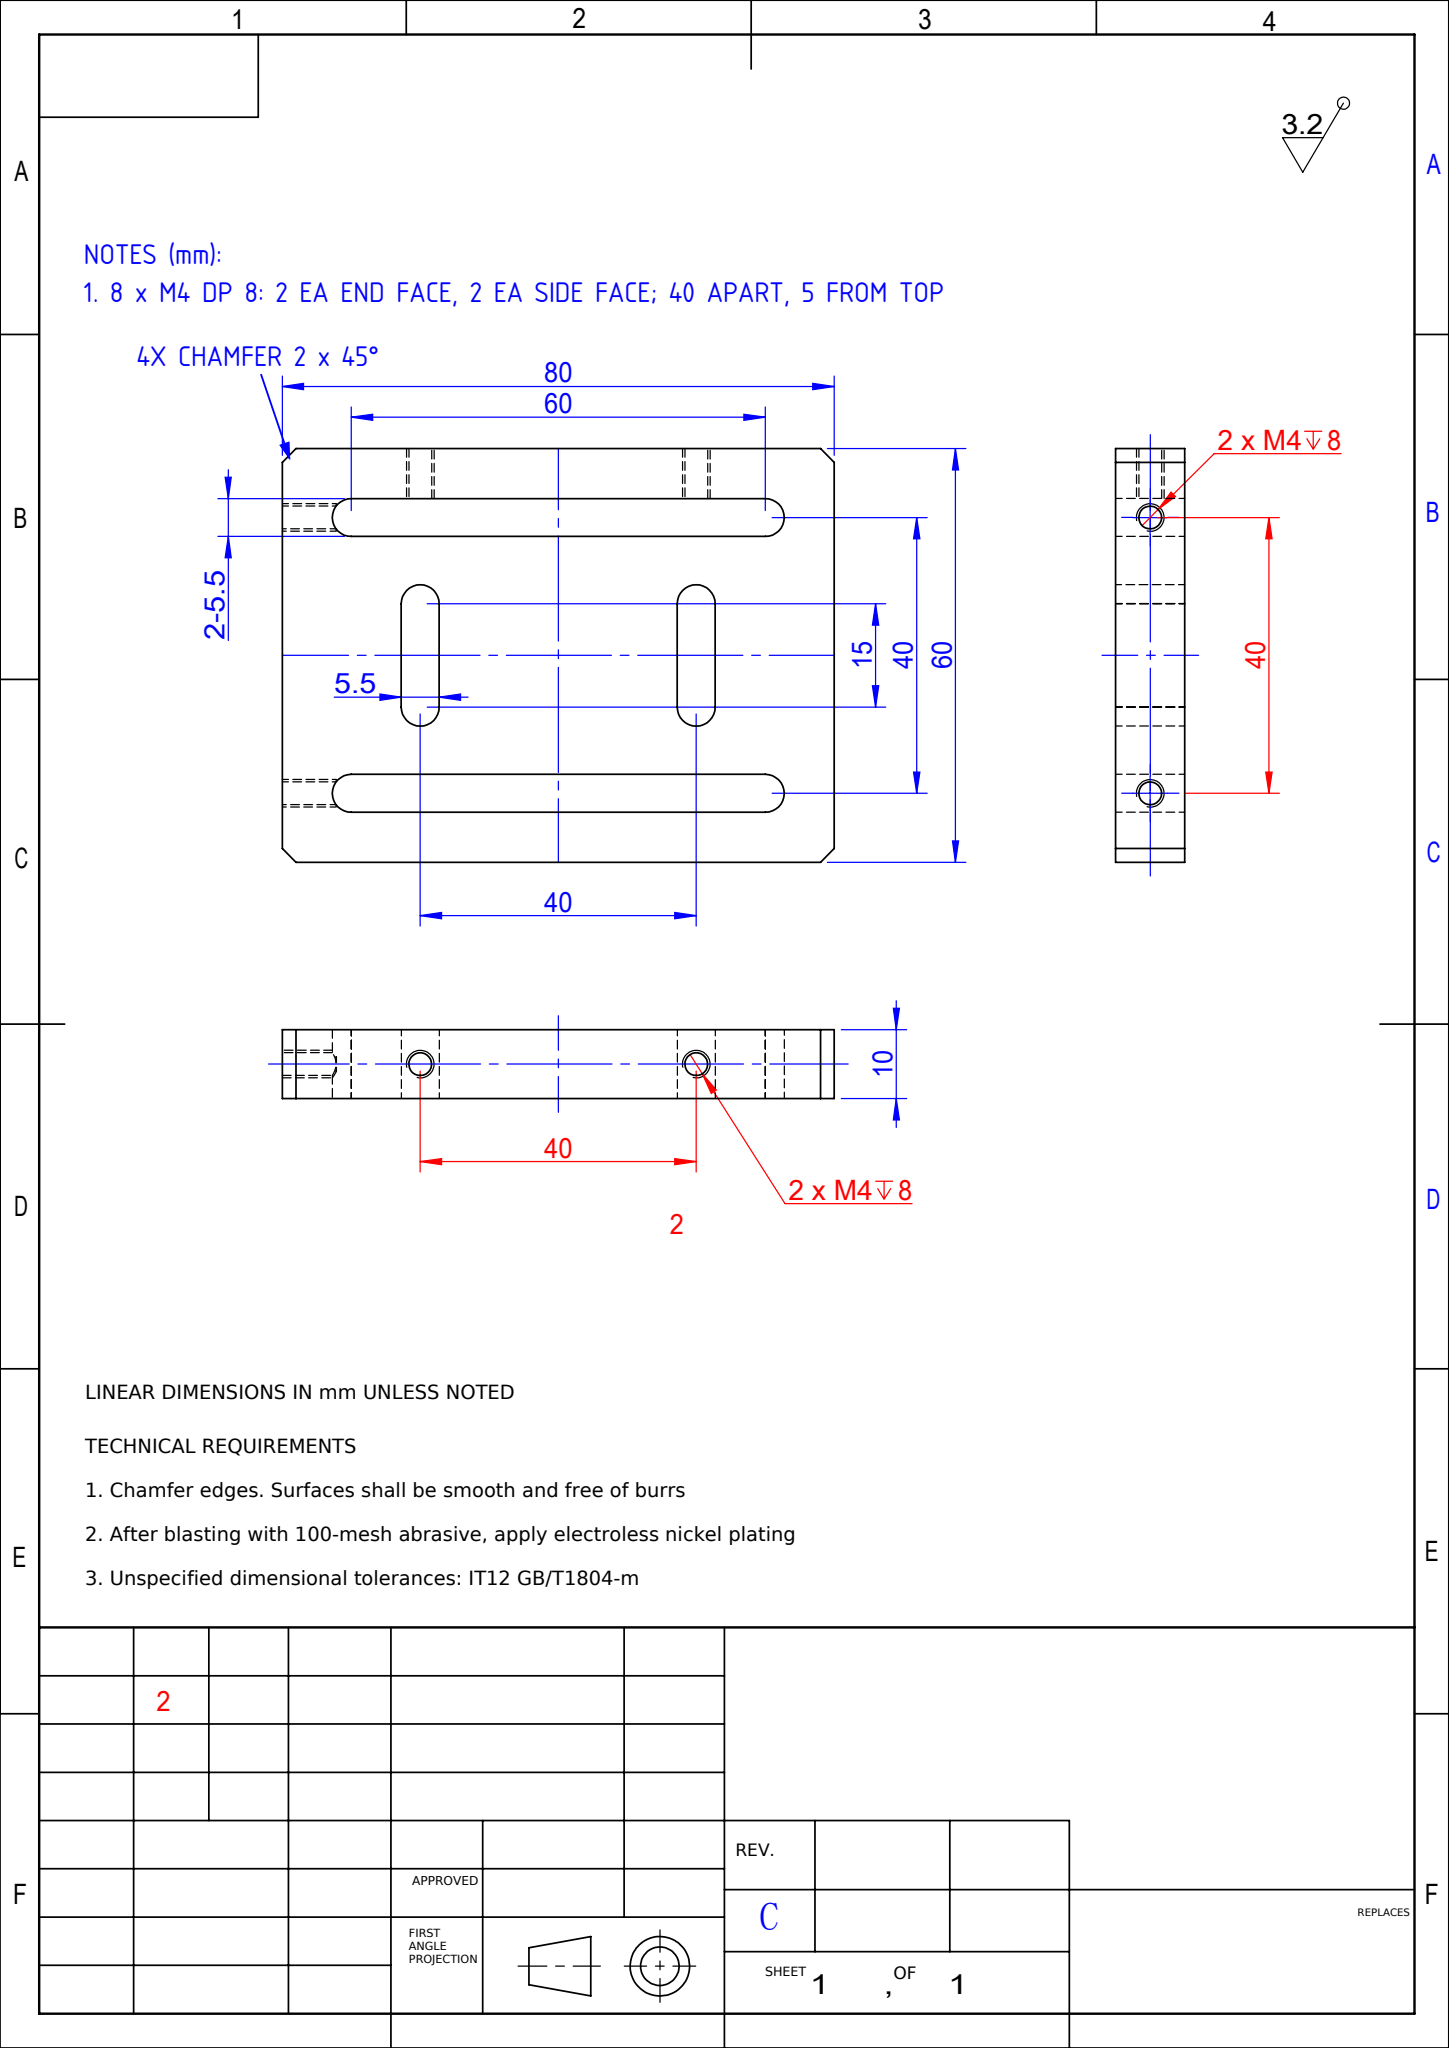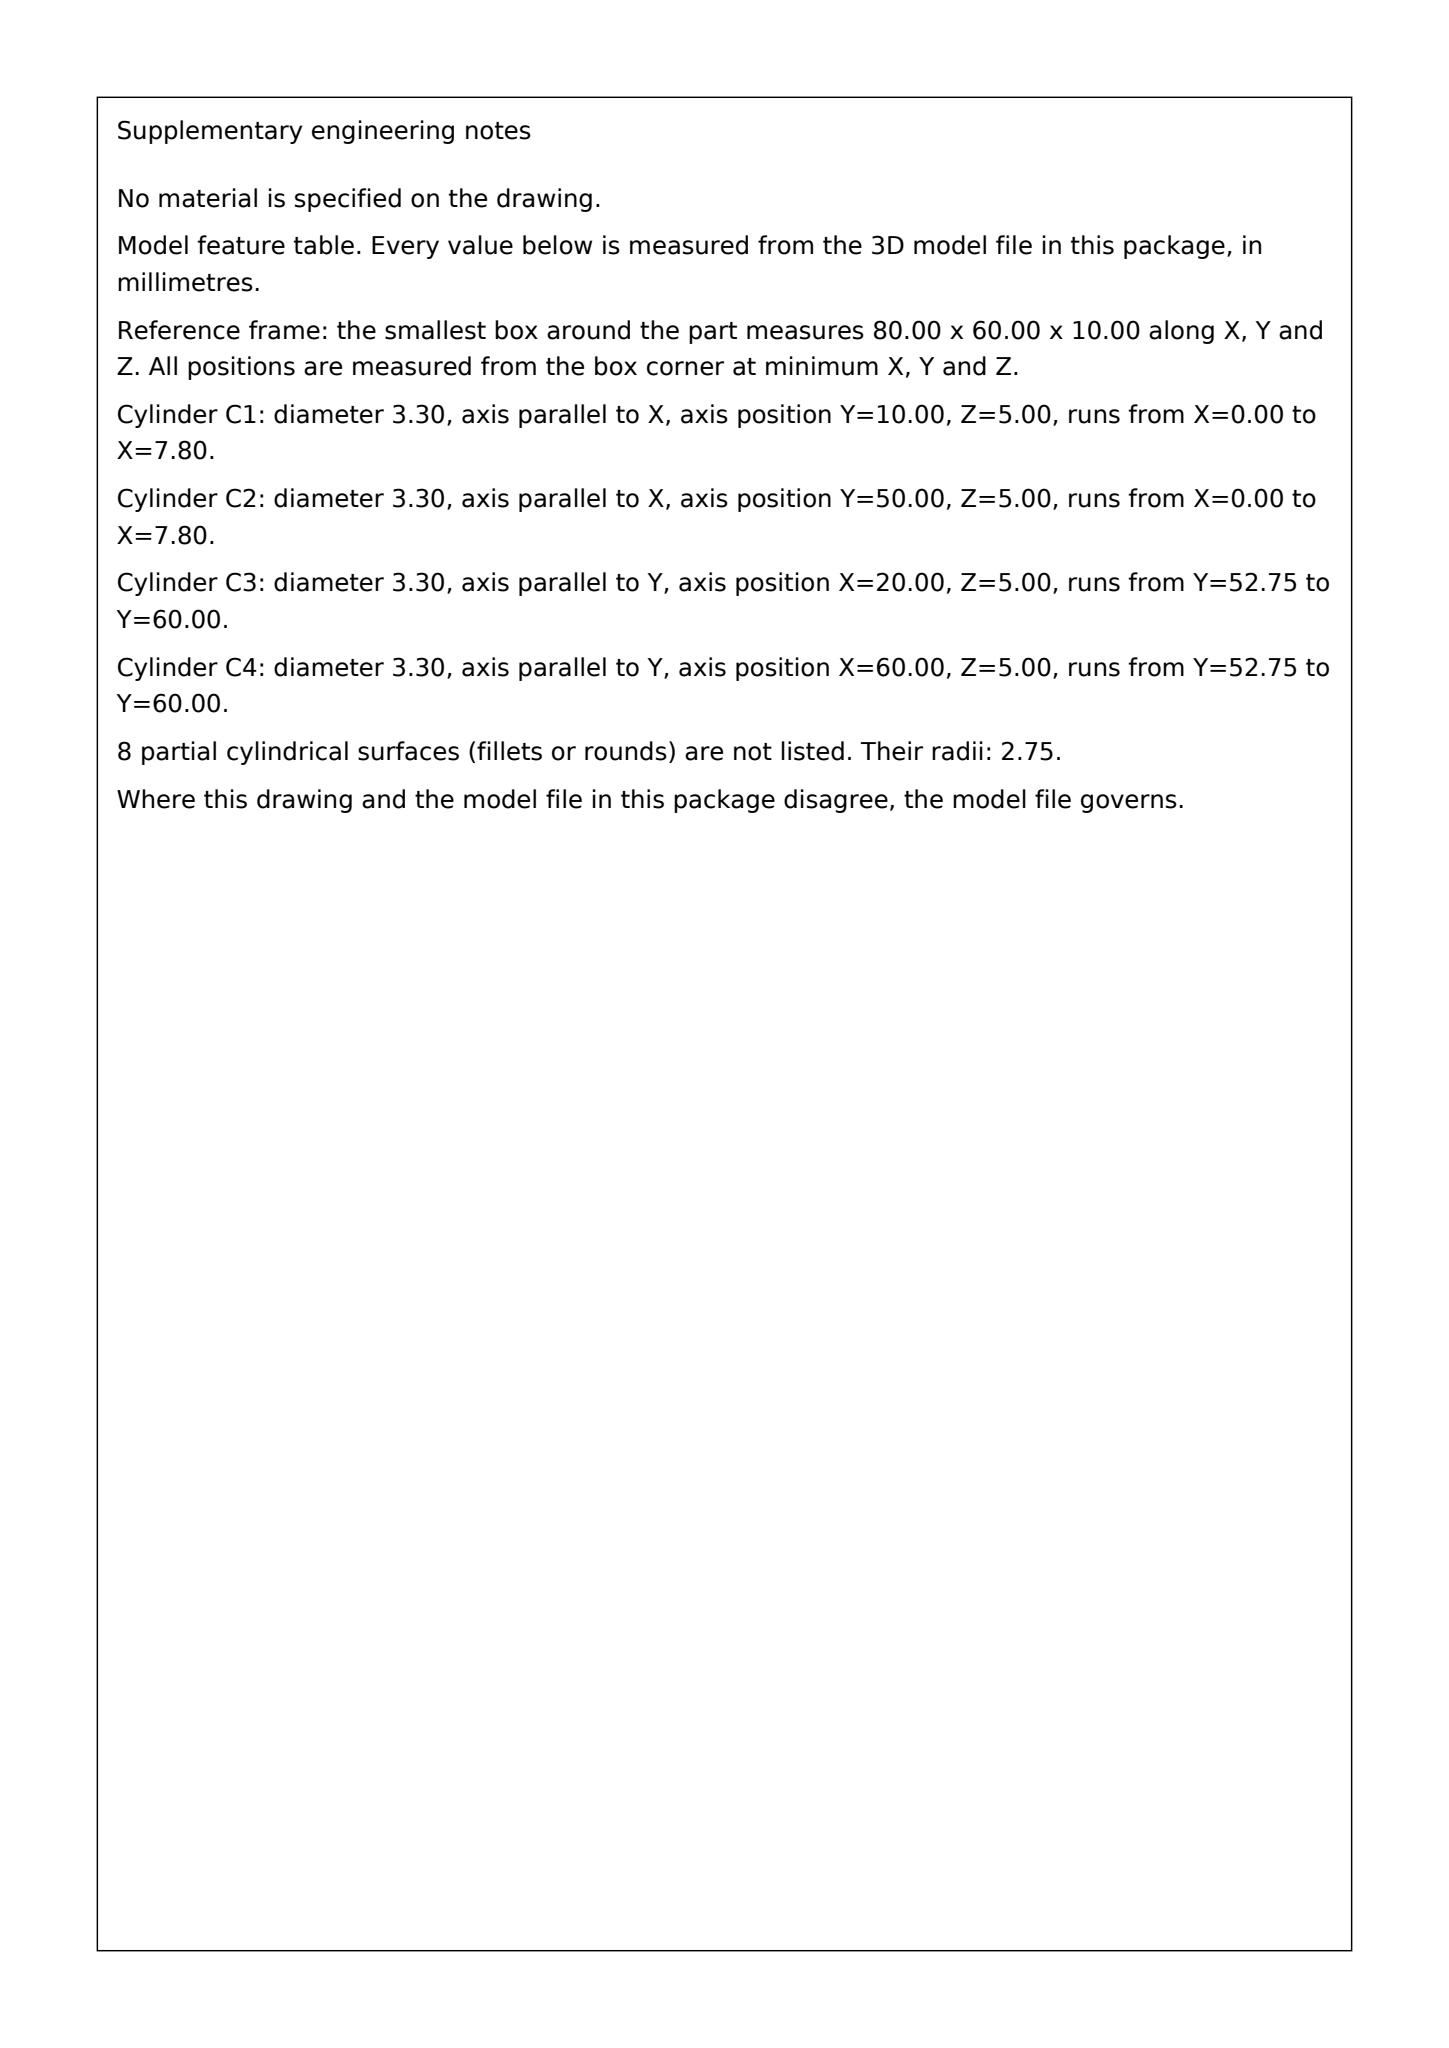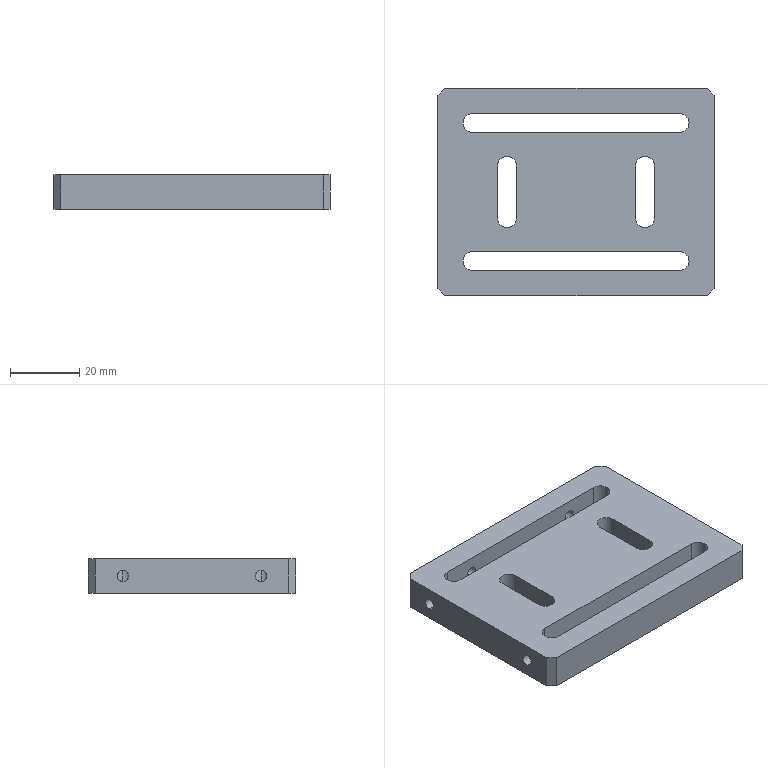Part | SolidWorks | mm | 1 solid | 36 faces | box 80 x 60 x 10 mm | volume 38469 mm3 | cylinder 18 | plane 18 | commonest cylinder face diameters 5.5 x10 3.3 x8
Drawing notes:
8 x M4 DP 8: 2 EA END FACE, 2 EA SIDE FACE; 40 APART, 5 FROM TOP | from the solid: 3.3 dia x-axis holes at (y=10,z=5) x2 and (y=50,z=5) x2, L=7.8; 3.3 dia y-axis holes at (x=20,z=5) x2 and (x=60,z=5) x2, L=7.25; bbox 80x60x10
4X CHAMFER 2 x 45° AT THE FOUR VERTICAL CORNERS OF THE 80 x 60 PLATE OUTLINE, FULL 10 THICKNESS | from the solid: inclined_planes: four 45°/45°/90° faces, size [2.0, 2.0, 10.0], at bbox corners [0,0,0], [0,58,0], [78,0,0], [78,58,0]
build123d program:
from build123d import *

# Parameters (mm, degrees)
SKETCH1_W             = 80
SKETCH1_H             = 60
BOSS_EXTRUDE1_DEPTH   = 10
CUT_EXTRUDE1_DEPTH    = 51.99
CHAMFER1_SIZE         = 2
CUT_EXTRUDE2_DEPTH    = 51.99
M4_TAPPED_HOLE1_D     = 3.3
M4_TAPPED_HOLE1_DEPTH = 11.5
M4_TAPPED_HOLE1_TIP   = 0.9914
M4_TAPPED_HOLE2_D     = 3.3
M4_TAPPED_HOLE2_DEPTH = 11.5
M4_TAPPED_HOLE2_TIP   = 0.9914


with BuildPart() as part:
    # Sketch1 → Boss-Extrude1 (new body)
    with BuildSketch(Plane.XY):
        Rectangle(SKETCH1_W, SKETCH1_H)
    extrude(amount=BOSS_EXTRUDE1_DEPTH)

    # Sketch2 → Cut-Extrude1 (cut, through all)
    with BuildSketch(Plane.XY.offset(10)):
        with BuildLine():
            Line((-30, 22.75), (30, 22.75))
            ThreePointArc((30, 22.75), (32.75, 20), (30, 17.25))
            Line((30, 17.25), (-30, 17.25))
            ThreePointArc((-30, 17.25), (-32.75, 20), (-30, 22.75))
        make_face()
        with BuildLine():
            Line((-30, -17.25), (30, -17.25))
            ThreePointArc((30, -17.25), (32.75, -20), (30, -22.75))
            Line((30, -22.75), (-30, -22.75))
            ThreePointArc((-30, -22.75), (-32.75, -20), (-30, -17.25))
        make_face()
    extrude(amount=-CUT_EXTRUDE1_DEPTH, mode=Mode.SUBTRACT)

    # Chamfer1
    chamfer1_edges = [part.edges().sort_by_distance(p)[0] for p in [
        (-40, 30, 5),
        (40, 30, 5),
        (40, -30, 5),
        (-40, -30, 5),
    ]]
    chamfer(chamfer1_edges, length=CHAMFER1_SIZE)

    # Sketch3 → Cut-Extrude2 (cut, through all)
    with BuildSketch(Plane.XY.offset(10)):
        with BuildLine():
            Line((-17.25, 7.5), (-17.25, -7.5))
            ThreePointArc((-17.25, -7.5), (-20, -10.25), (-22.75, -7.5))
            Line((-22.75, -7.5), (-22.75, 7.5))
            ThreePointArc((-22.75, 7.5), (-20, 10.25), (-17.25, 7.5))
        make_face()
        with BuildLine():
            Line((22.75, 7.5), (22.75, -7.5))
            ThreePointArc((22.75, -7.5), (20, -10.25), (17.25, -7.5))
            Line((17.25, -7.5), (17.25, 7.5))
            ThreePointArc((17.25, 7.5), (20, 10.25), (22.75, 7.5))
        make_face()
    extrude(amount=-CUT_EXTRUDE2_DEPTH, mode=Mode.SUBTRACT)

    # M4 Tapped Hole1
    with Locations(Plane(origin=(-40, 18.994, -6.093), x_dir=(0, 0, -1), z_dir=(-1, 0, 0))):
        with Locations((-11.093, -1.006), (-11.093, 38.994)):
            Hole(M4_TAPPED_HOLE1_D / 2, depth=M4_TAPPED_HOLE1_DEPTH)
            with Locations((0, 0, -(M4_TAPPED_HOLE1_DEPTH + M4_TAPPED_HOLE1_TIP / 2))):  # 118° drill point
                Cone(0, M4_TAPPED_HOLE1_D / 2, M4_TAPPED_HOLE1_TIP, mode=Mode.SUBTRACT)

    # M4 Tapped Hole2
    with Locations(Plane(origin=(0, 30, 0), x_dir=(-1, 0, 0), z_dir=(0, 1, 0))):
        with Locations((20, 5), (-20, 5)):
            Hole(M4_TAPPED_HOLE2_D / 2, depth=M4_TAPPED_HOLE2_DEPTH)
            with Locations((0, 0, -(M4_TAPPED_HOLE2_DEPTH + M4_TAPPED_HOLE2_TIP / 2))):  # 118° drill point
                Cone(0, M4_TAPPED_HOLE2_D / 2, M4_TAPPED_HOLE2_TIP, mode=Mode.SUBTRACT)


solid = part.part